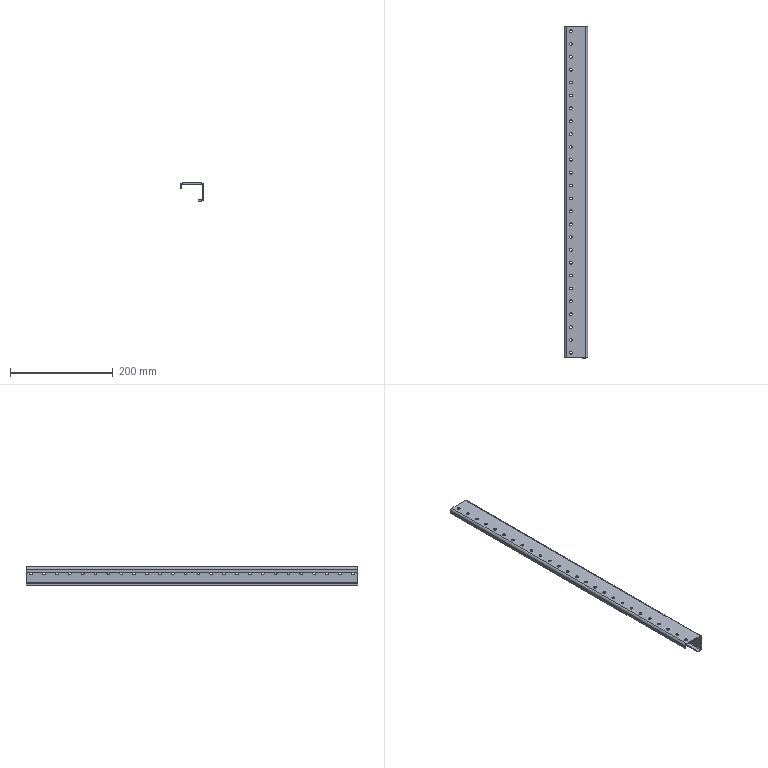Component | SolidWorks | BottomSideBeam-1 | 1 solid | 134 faces | volume 113895 mm3 | cylinder 110 | plane 24 | commonest cylinder face diameters 5.4 x104 4 x3 8 x3